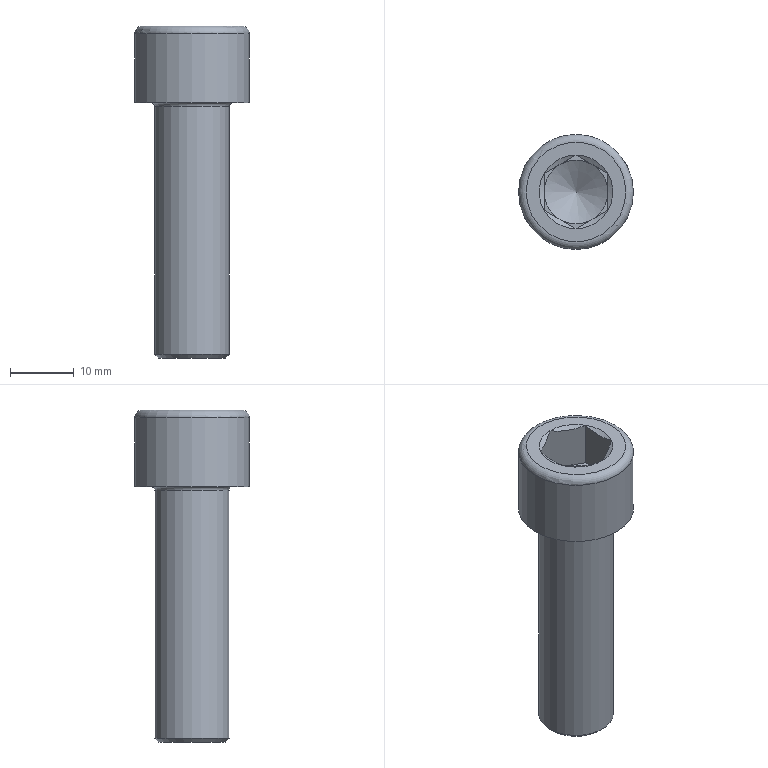Component | NX | GB-T70_1-2000_M12X40 | 1 solid | 27 faces | volume 6632 mm3 | plane 15 | cone 8 | cylinder 2 | torus 2 | commonest cylinder face diameters 11.701 x1 18 x1